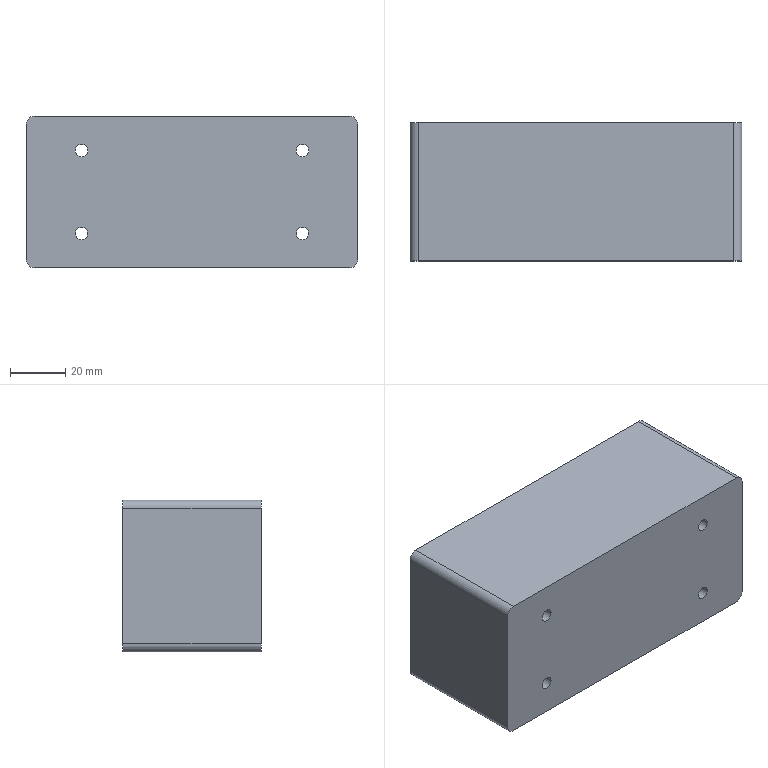CAM job | Mastercam | mm | 10 operations | part box 120 x 50 x 55
1. Facing | 24 - 100 平铣刀
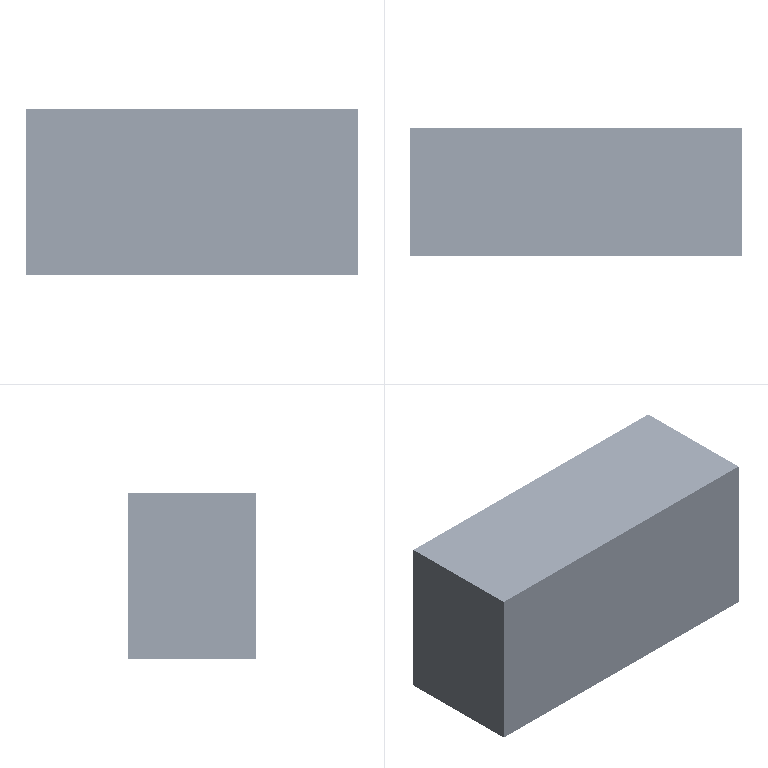2. Contour (Ramp) | 20 - 20 平铣刀
3. Contour (2D) | 20 - 20 平铣刀
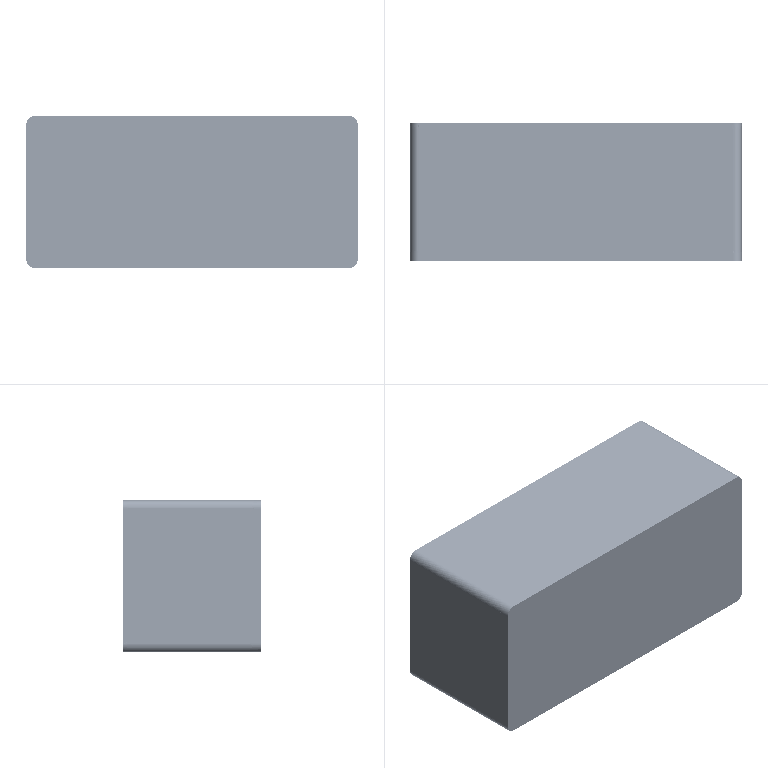4. Contour (Ramp) | 5 - 5 平铣刀
5. Contour (2D) | 5 - 5 平铣刀
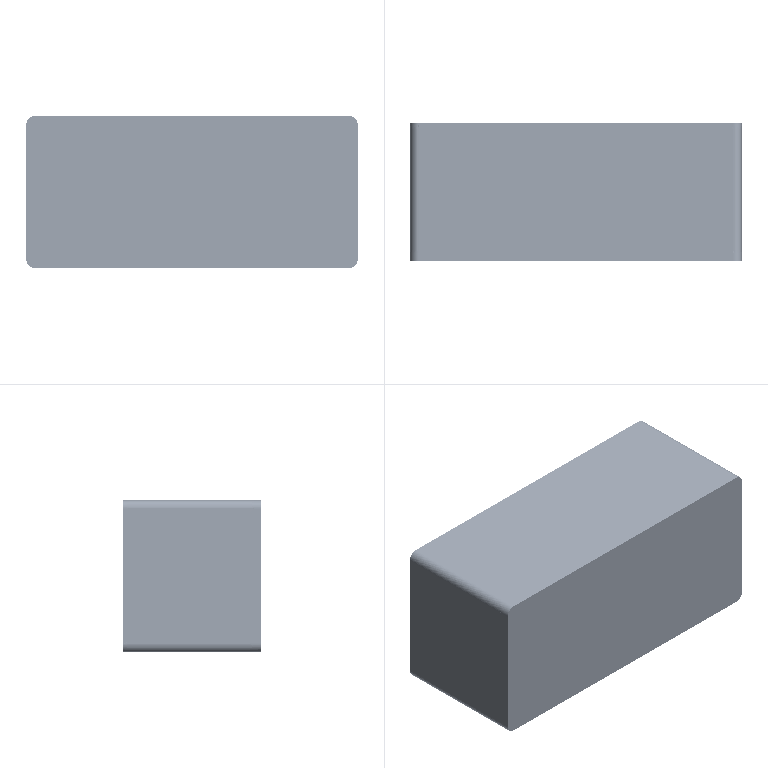6. Drill/Counterbore | 7 - 4 倒角刀
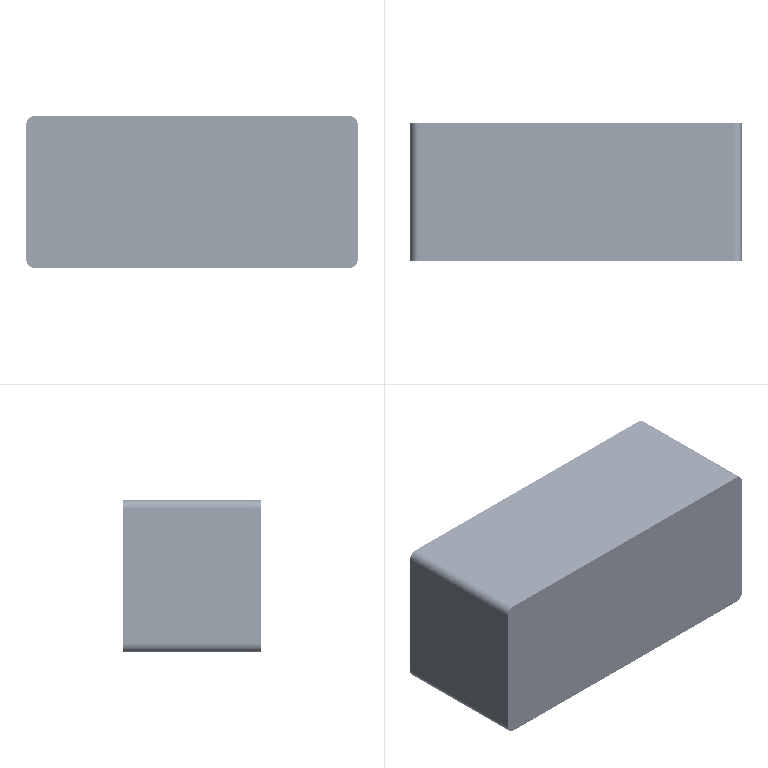7. Contour (2D chamfer) | 7 - 4 倒角刀
8. Facing | 24 - 100 平铣刀
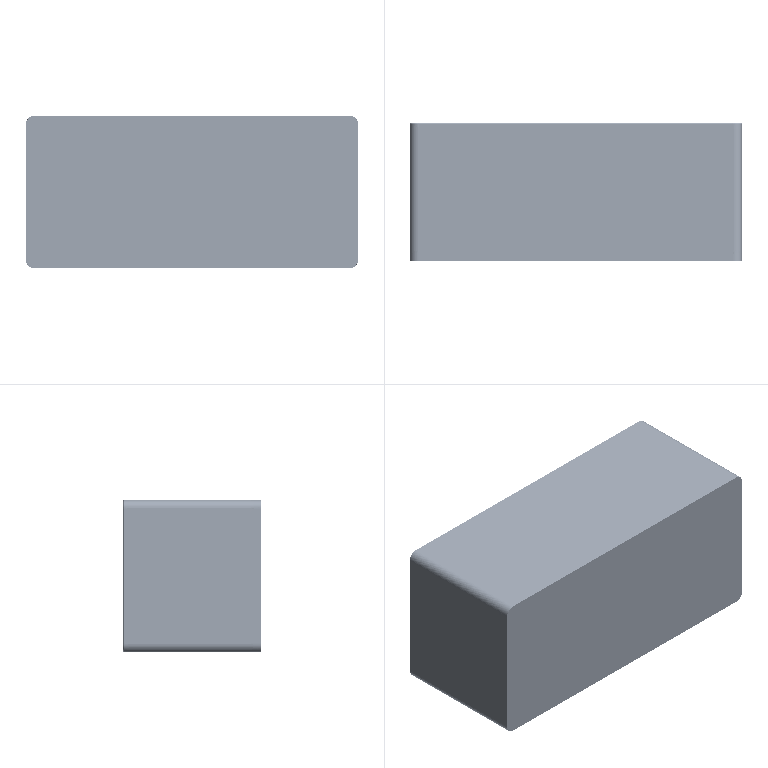9. Drill/Counterbore | 7 - 4 倒角刀
10. Contour (2D chamfer) | 7 - 4 倒角刀